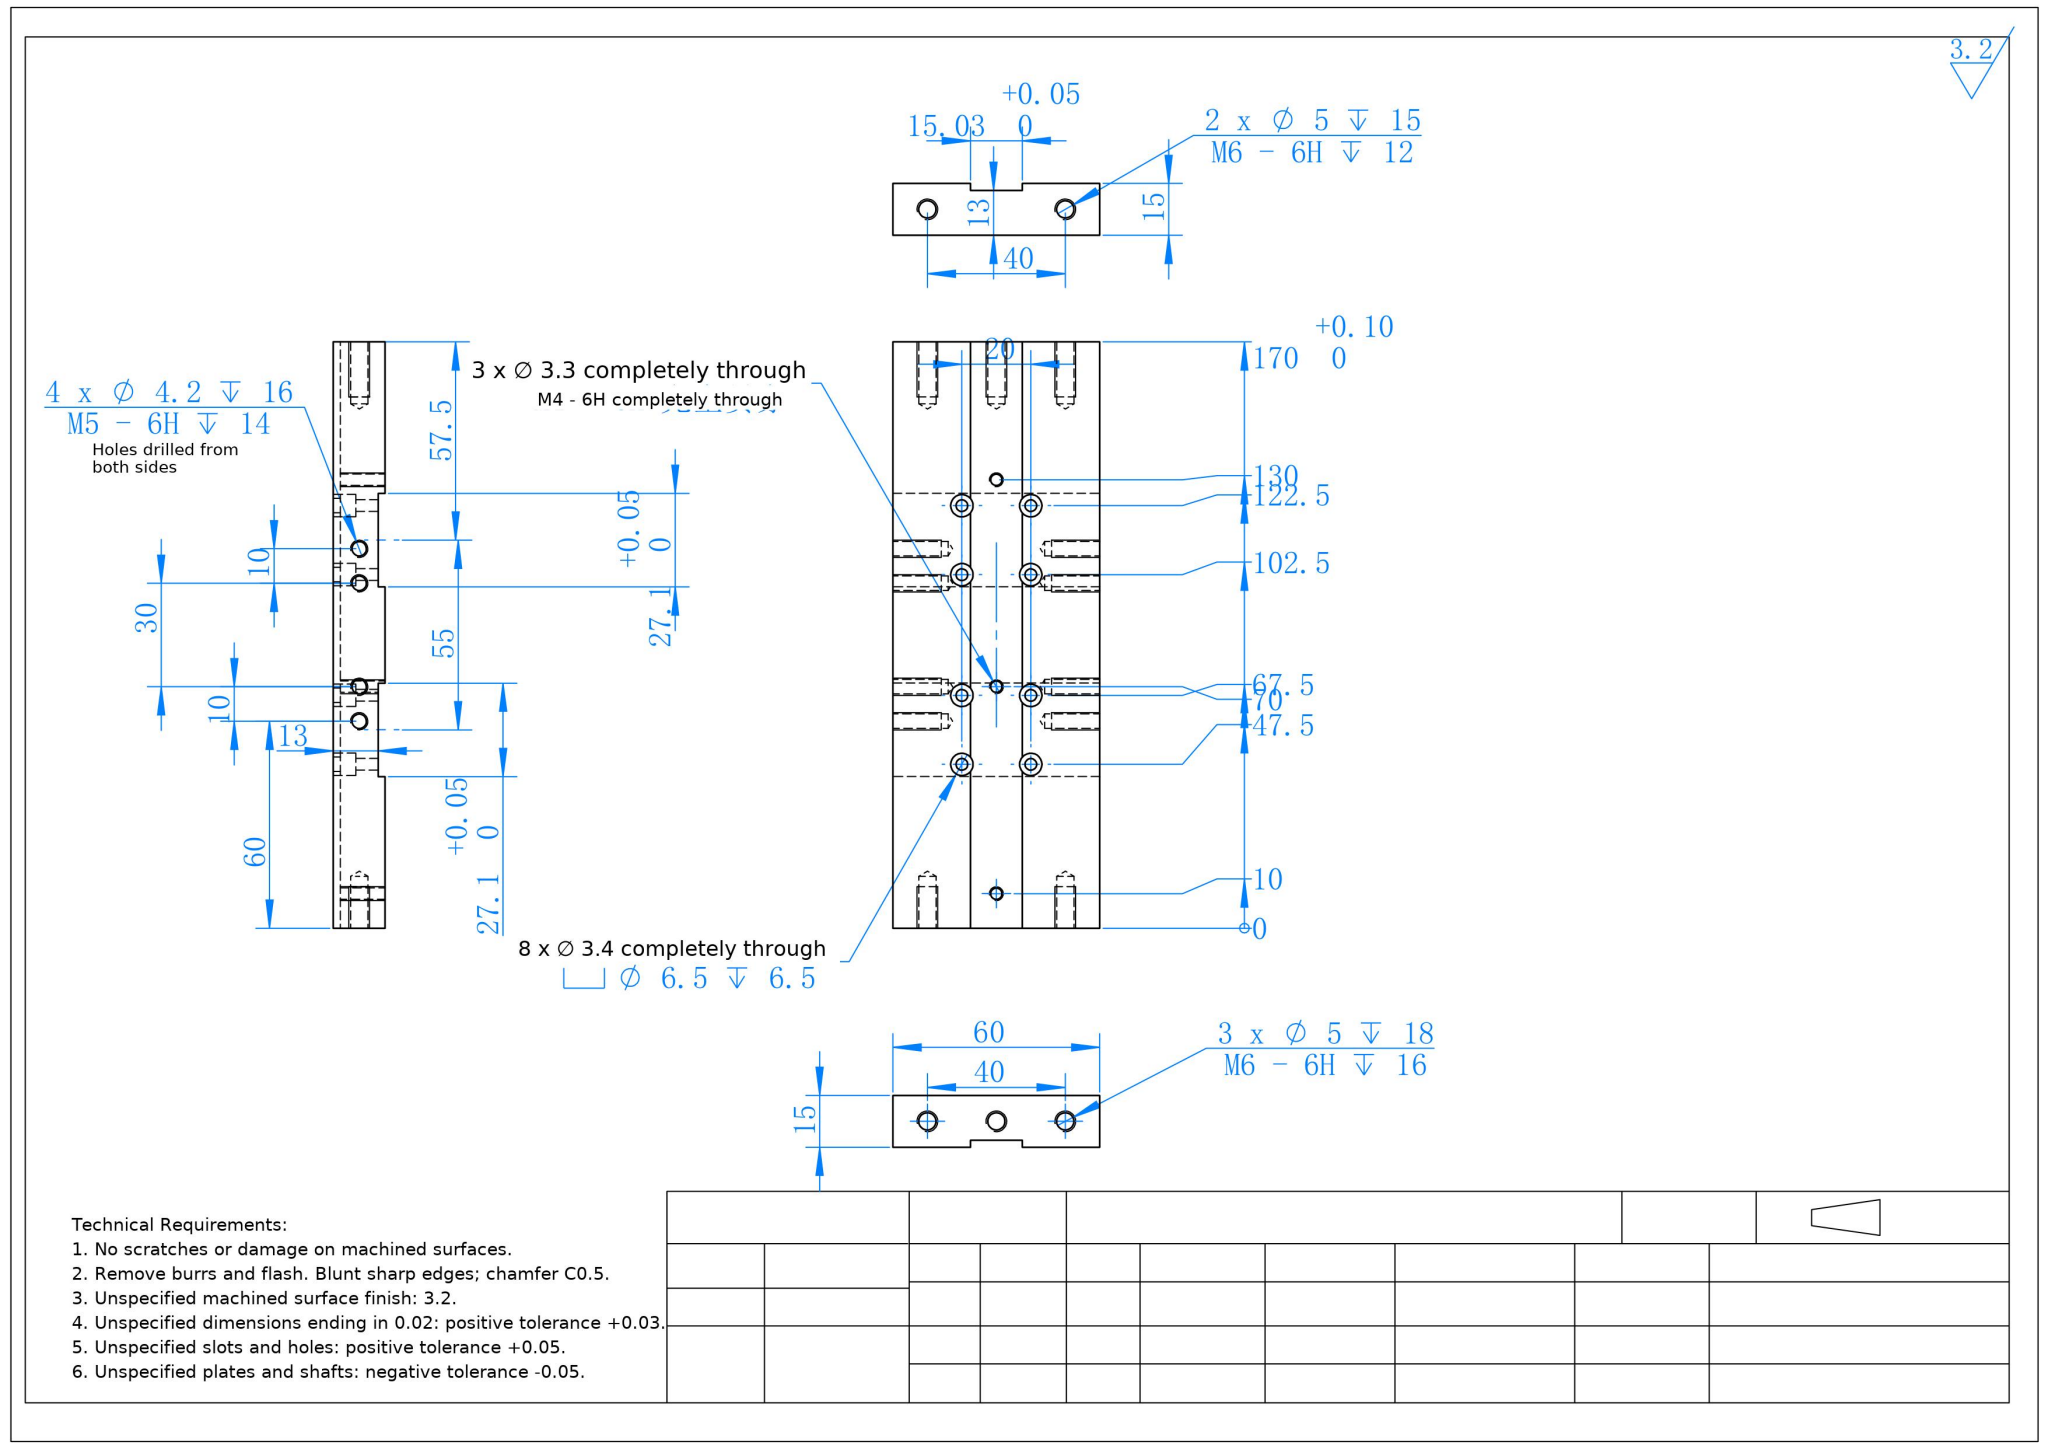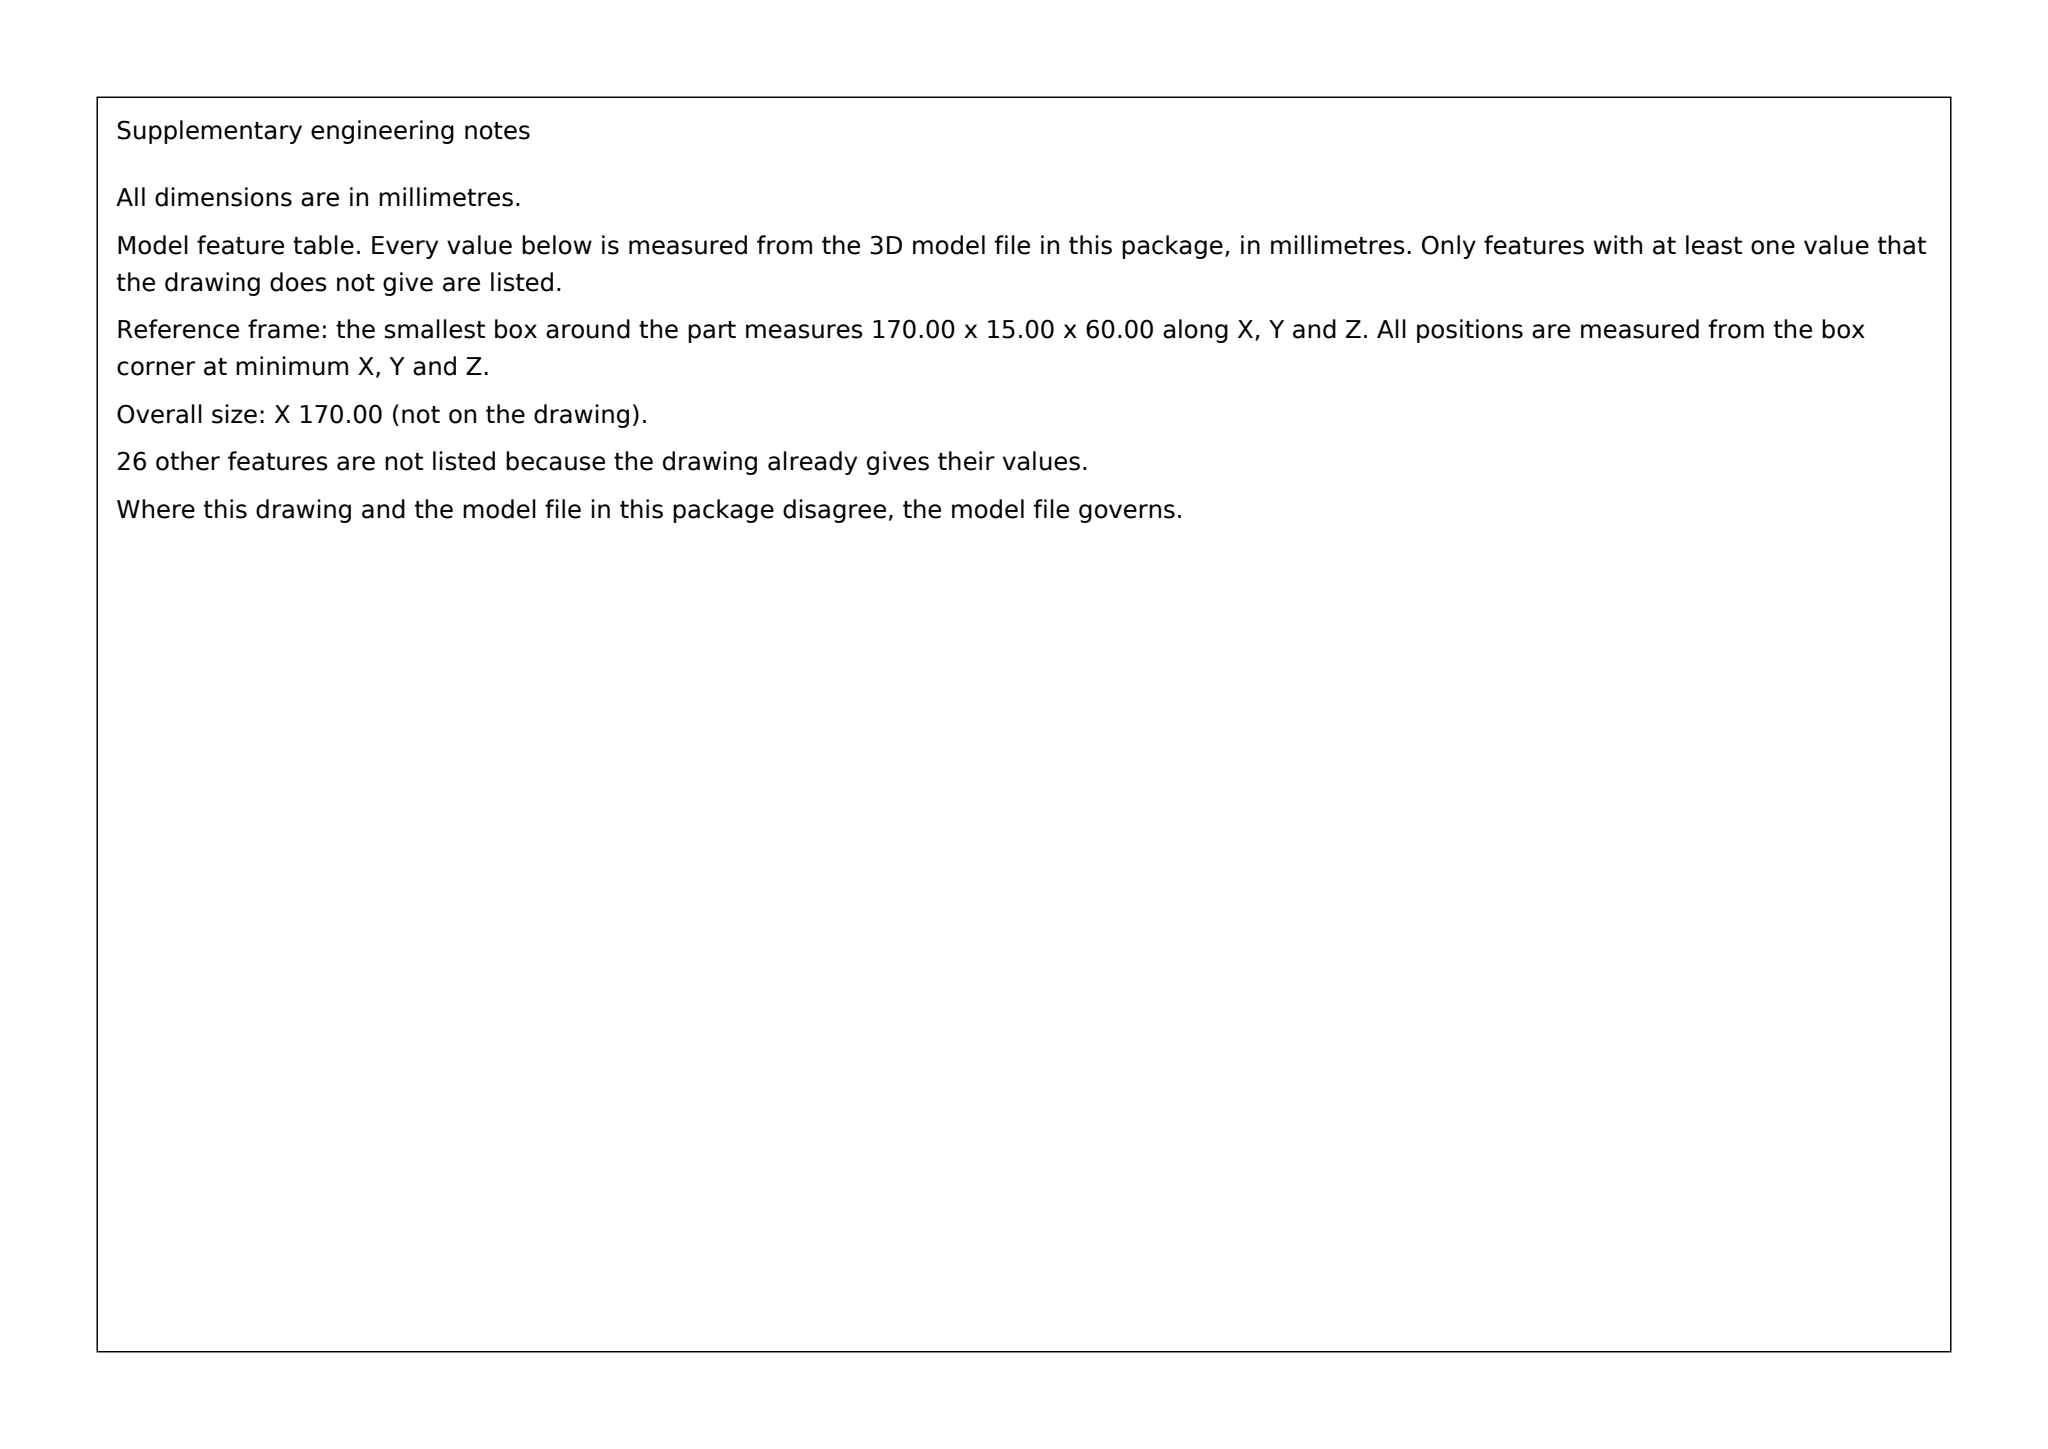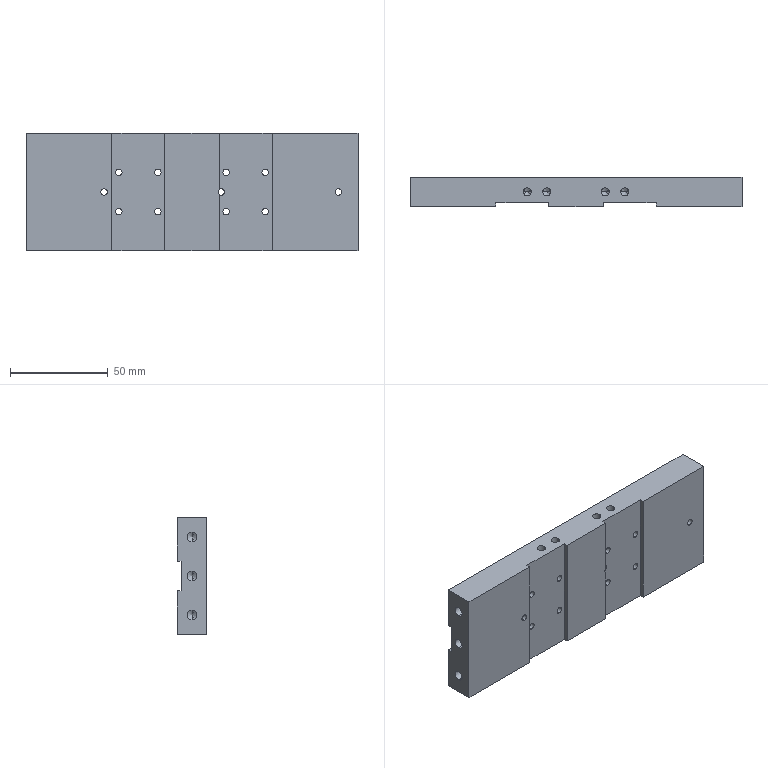Part | SolidWorks | mm | 1 solid | 125 faces | box 170 x 15 x 60 mm | volume 135386 mm3 | cylinder 64 | plane 35 | cone 26 | commonest cylinder face diameters 4.2 x16 3.4 x16 6.5 x16 5 x10 3.3 x6
build123d program:
from build123d import *

# Parameters (mm, degrees)
SKETCH1_W                                       = 170
SKETCH1_H                                       = 15
EXTRUDE1_DEPTH                                  = 30
SKETCH20_W                                      = 170
SKETCH20_H                                      = 15.03
CUT_EXTRUDE3_DEPTH                              = 2
SKETCH31_W                                      = 27.1
SKETCH31_H                                      = 60
CUT_EXTRUDE4_DEPTH                              = 2
M6_TAPPED_HOLE2_D                               = 5
M6_TAPPED_HOLE2_DEPTH                           = 18
M6_TAPPED_HOLE2_TIP                             = 1.502
M4_TAPPED_HOLE1_D                               = 3.3
M3_HEX_SOCKET_HEAD_CAP_SCREW_CBORE1_D           = 3.4
M3_HEX_SOCKET_HEAD_CAP_SCREW_CBORE1_CBORE_D     = 6.5
M3_HEX_SOCKET_HEAD_CAP_SCREW_CBORE1_CBORE_DEPTH = 6.5
M6_TAPPED_HOLE1_D                               = 5
M6_TAPPED_HOLE1_DEPTH                           = 15
M6_TAPPED_HOLE1_TIP                             = 1.502
M5_TAPPED_HOLE1_D                               = 4.2
M5_TAPPED_HOLE1_DEPTH                           = 16
M5_TAPPED_HOLE1_TIP                             = 1.262
M5_TAPPED_HOLE3_D                               = 4.2
M5_TAPPED_HOLE3_DEPTH                           = 16
M5_TAPPED_HOLE3_TIP                             = 1.262


with BuildPart() as part:
    # Sketch1 → Extrude1 (new, symmetric)
    with BuildSketch(Plane.XY):
        Rectangle(SKETCH1_W, SKETCH1_H)
    extrude(amount=EXTRUDE1_DEPTH, both=True)

    # Sketch20 → Cut-Extrude3 (cut)
    with BuildSketch(Plane(origin=(0, 7.5, 0), x_dir=(-1, 0, 0), z_dir=(0, 1, 0))):
        Rectangle(SKETCH20_W, SKETCH20_H)
    extrude(amount=-CUT_EXTRUDE3_DEPTH, mode=Mode.SUBTRACT)

    # Sketch31 → Cut-Extrude4 (cut)
    with BuildSketch(Plane(origin=(0, -7.5, 0), x_dir=(-1, 0, 0), z_dir=(0, -1, 0))):
        with Locations((27.5, 0)):
            Rectangle(SKETCH31_W, SKETCH31_H)
        with Locations((-27.5, 0)):
            Rectangle(SKETCH31_W, SKETCH31_H)
    extrude(amount=-CUT_EXTRUDE4_DEPTH, mode=Mode.SUBTRACT)

    # M6 Tapped Hole2
    with Locations(Plane.ZY.offset(85)):
        with Locations((-20, 0), (20, 0), (0, 0)):
            Hole(M6_TAPPED_HOLE2_D / 2, depth=M6_TAPPED_HOLE2_DEPTH)
            with Locations((0, 0, -(M6_TAPPED_HOLE2_DEPTH + M6_TAPPED_HOLE2_TIP / 2))):  # 118° drill point
                Cone(0, M6_TAPPED_HOLE2_D / 2, M6_TAPPED_HOLE2_TIP, mode=Mode.SUBTRACT)

    # M4 Tapped Hole1 (through all)
    with Locations(Plane(origin=(0, 7.5, 0), x_dir=(1, 0, 0), z_dir=(0, 1, 0))):
        with Locations((15, 0), (75, 0), (-45, 0)):
            Hole(M4_TAPPED_HOLE1_D / 2)

    # M3 Hex Socket Head Cap Screw CBORE1 (through all)
    with Locations(Plane(origin=(0, 7.5, 0), x_dir=(1, 0, 0), z_dir=(0, 1, 0))):
        with Locations((-37.5, 10), (-17.5, 10), (-37.5, -10), (-17.5, -10), (17.5, 10), (37.5, 10), (17.5, -10), (37.5, -10)):
            CounterBoreHole(M3_HEX_SOCKET_HEAD_CAP_SCREW_CBORE1_D / 2, M3_HEX_SOCKET_HEAD_CAP_SCREW_CBORE1_CBORE_D / 2, M3_HEX_SOCKET_HEAD_CAP_SCREW_CBORE1_CBORE_DEPTH)

    # M6 Tapped Hole1
    with Locations(Plane(origin=(85, 0, 0), x_dir=(0, 0, -1), z_dir=(1, 0, 0))):
        with Locations((-20, 0), (20, 0)):
            Hole(M6_TAPPED_HOLE1_D / 2, depth=M6_TAPPED_HOLE1_DEPTH)
            with Locations((0, 0, -(M6_TAPPED_HOLE1_DEPTH + M6_TAPPED_HOLE1_TIP / 2))):  # 118° drill point
                Cone(0, M6_TAPPED_HOLE1_D / 2, M6_TAPPED_HOLE1_TIP, mode=Mode.SUBTRACT)

    # M5 Tapped Hole1
    with Locations(Plane(origin=(0, 0, -30), x_dir=(1, 0, 0), z_dir=(0, 0, -1))):
        with Locations((-15, 0), (15, 0), (25, 0), (-25, 0)):
            Hole(M5_TAPPED_HOLE1_D / 2, depth=M5_TAPPED_HOLE1_DEPTH)
            with Locations((0, 0, -(M5_TAPPED_HOLE1_DEPTH + M5_TAPPED_HOLE1_TIP / 2))):  # 118° drill point
                Cone(0, M5_TAPPED_HOLE1_D / 2, M5_TAPPED_HOLE1_TIP, mode=Mode.SUBTRACT)

    # M5 Tapped Hole3
    with Locations(Plane.XY.offset(30)):
        with Locations((15, 0), (-15, 0), (-25, 0), (25, 0)):
            Hole(M5_TAPPED_HOLE3_D / 2, depth=M5_TAPPED_HOLE3_DEPTH)
            with Locations((0, 0, -(M5_TAPPED_HOLE3_DEPTH + M5_TAPPED_HOLE3_TIP / 2))):  # 118° drill point
                Cone(0, M5_TAPPED_HOLE3_D / 2, M5_TAPPED_HOLE3_TIP, mode=Mode.SUBTRACT)


solid = part.part